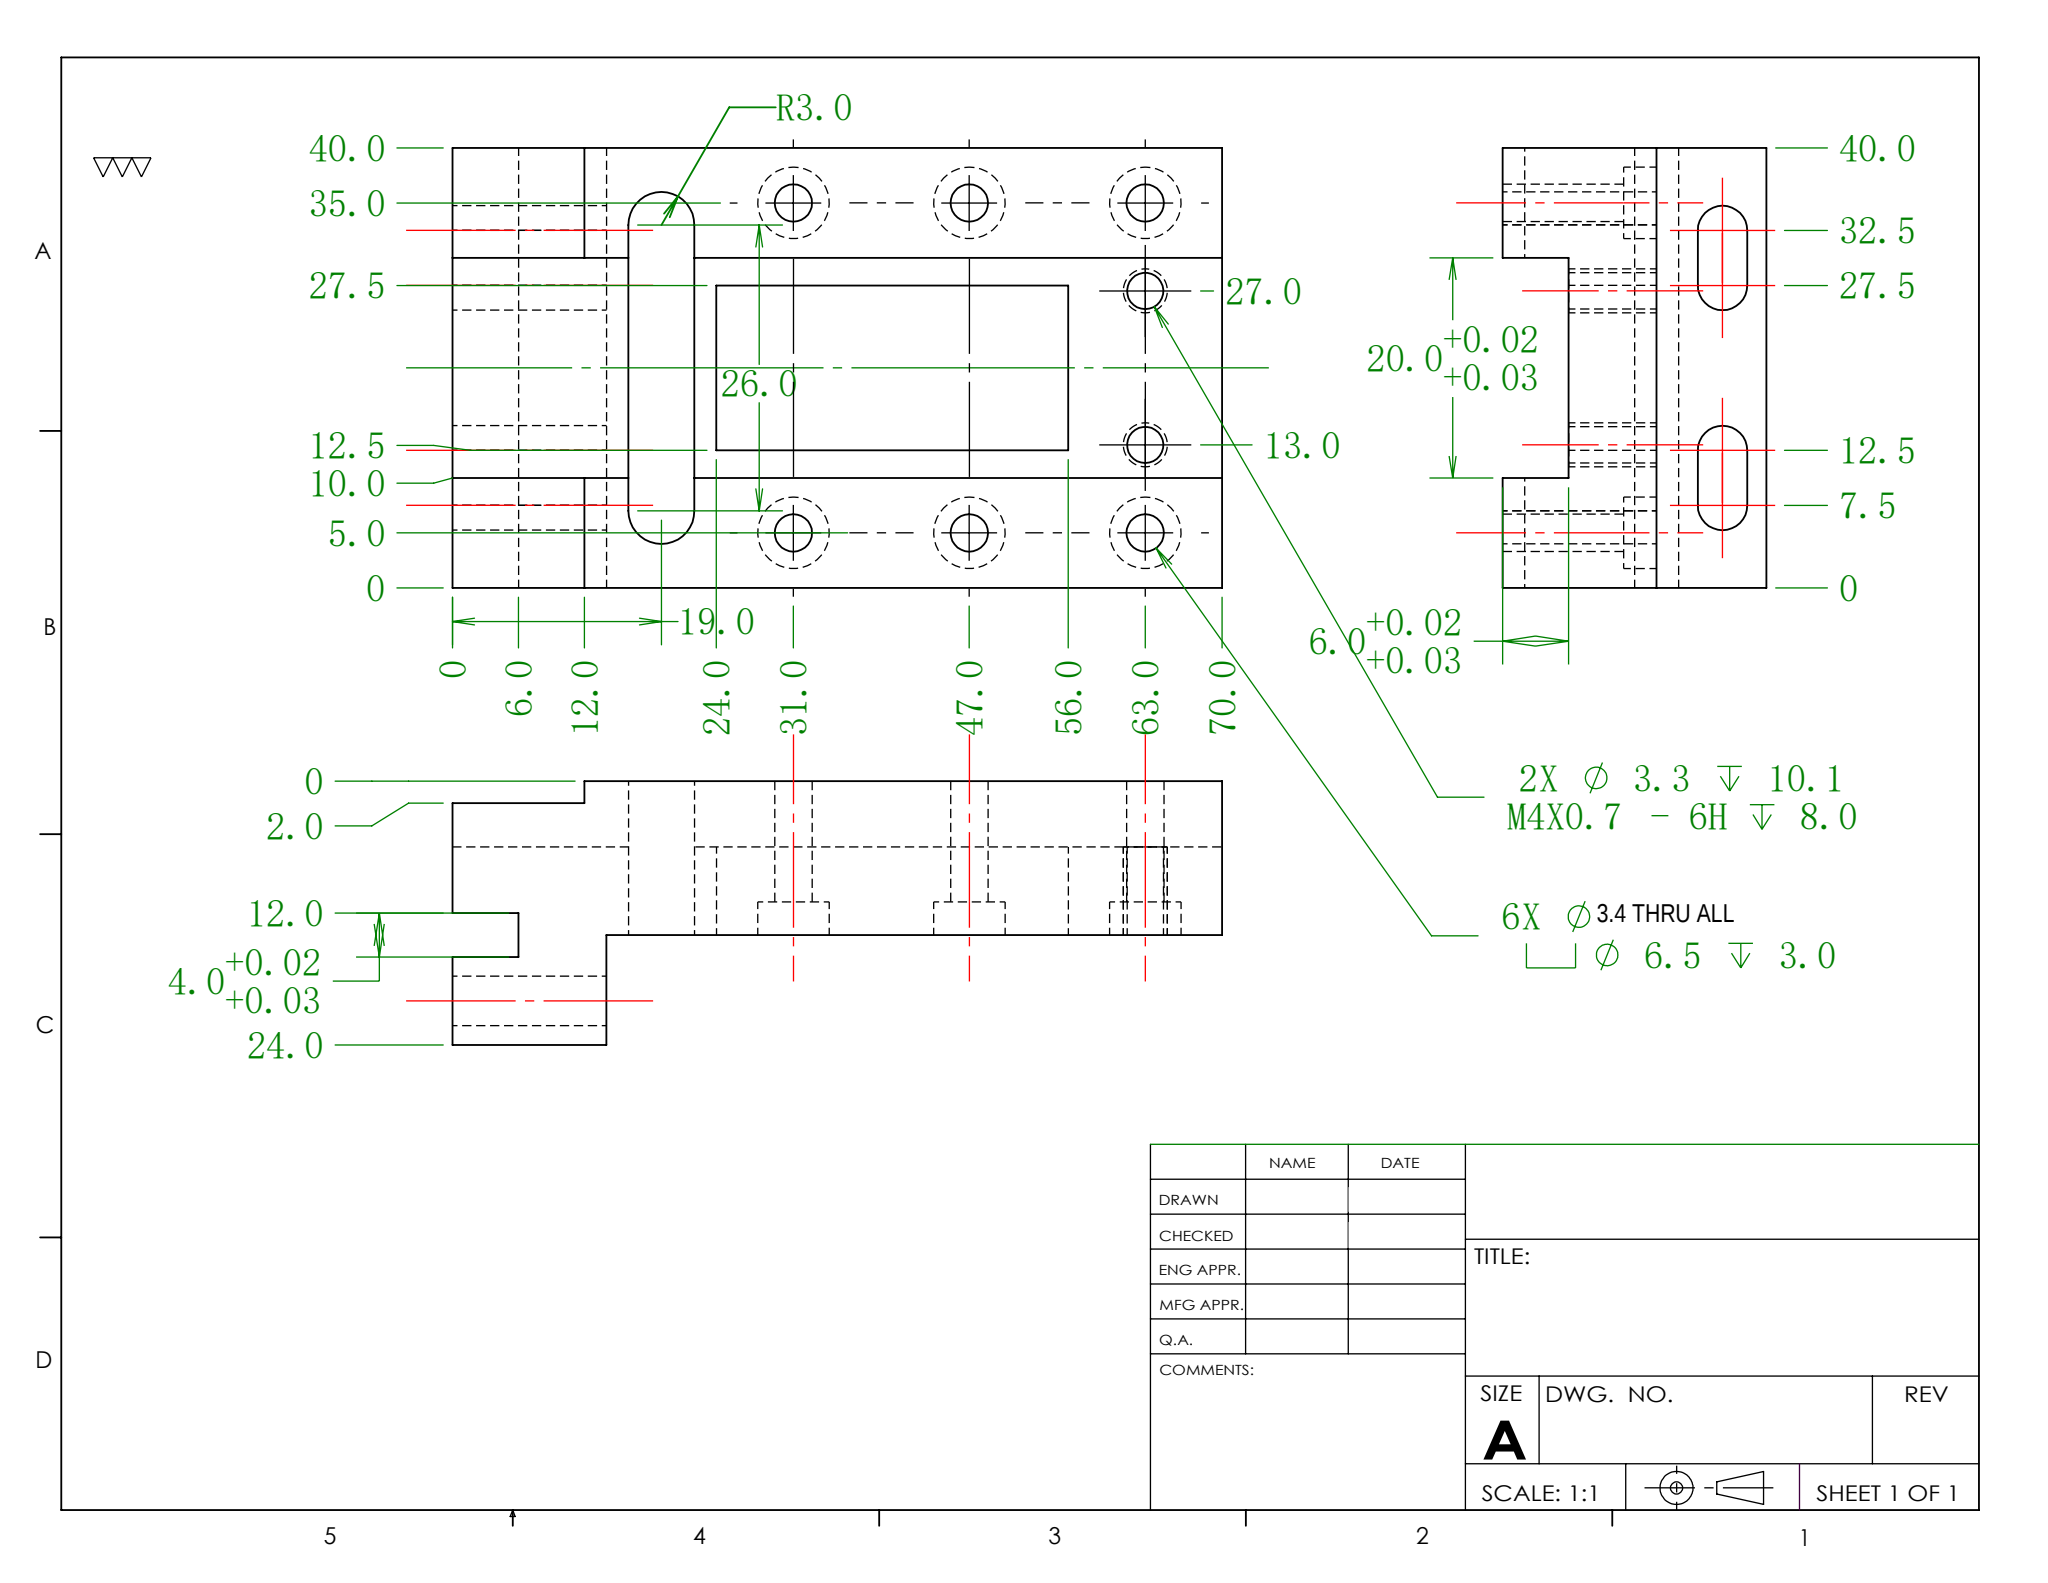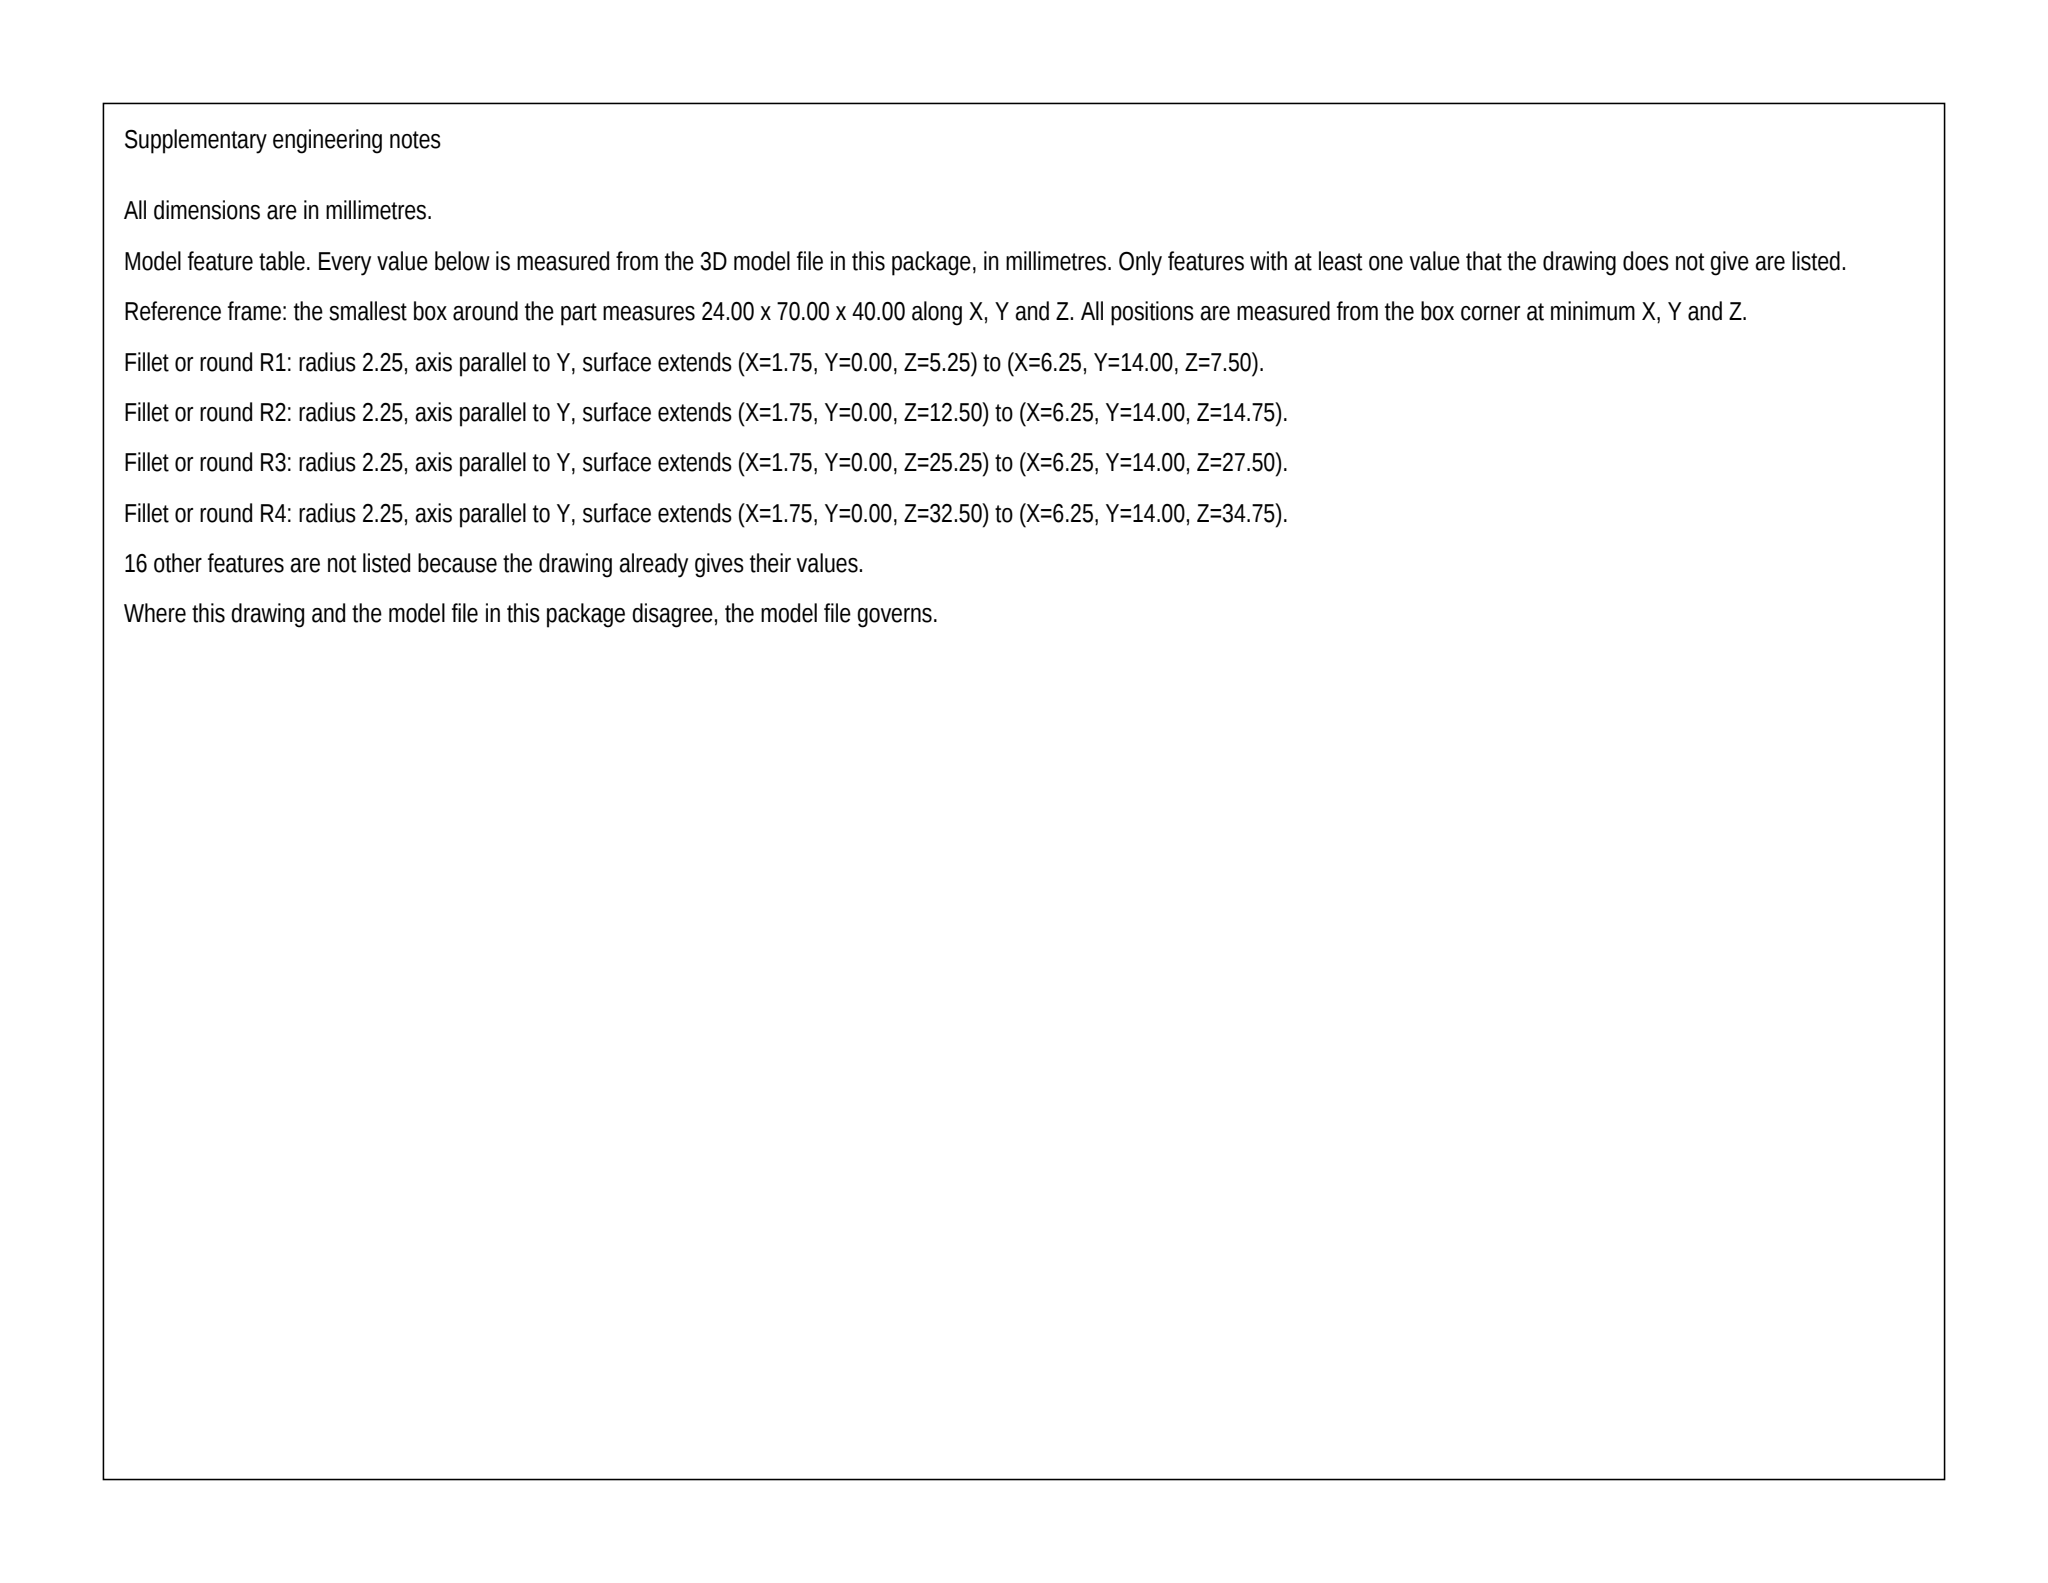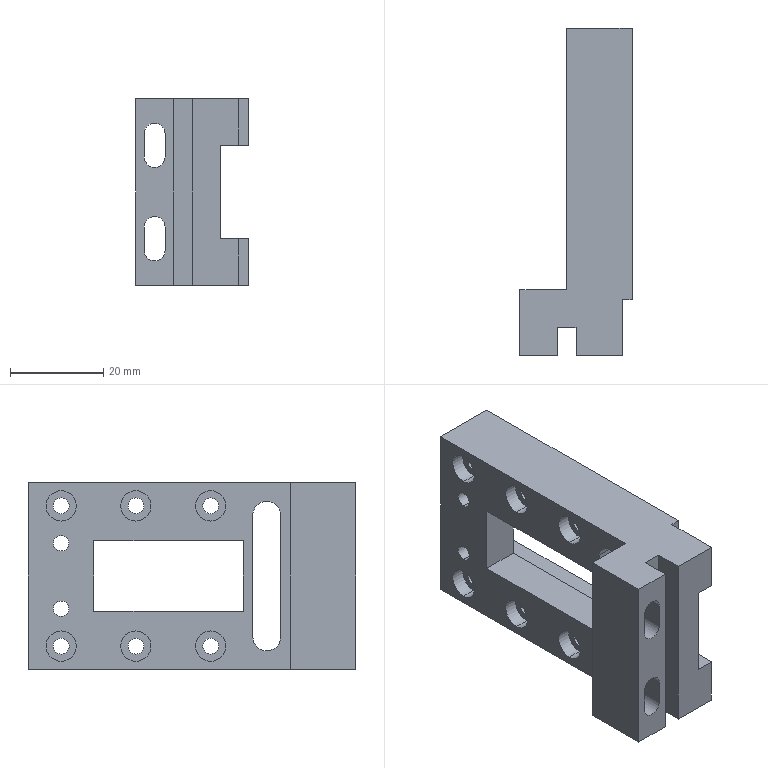Part | SolidWorks | mm | 1 solid | 76 faces | box 24 x 70 x 40 mm | volume 26851 mm3 | plane 39 | cylinder 37 | commonest cylinder face diameters 6.5 x12 3.4 x12 4.5 x6 3.3 x4 6 x3
build123d program:
from build123d import *

# Parameters (mm, degrees)
SKETCH1_W                                            = 40
SKETCH1_H                                            = 70
EXTRUDE1_DEPTH                                       = 12
SKETCH2_W                                            = 20
SKETCH2_H                                            = 80
EXTRUDE2_DEPTH                                       = 6
SKETCH3_W                                            = 40
SKETCH3_H                                            = 14
EXTRUDE3_DEPTH                                       = 12
SKETCH4_W                                            = 4
SKETCH4_H                                            = 6
EXTRUDE4_DEPTH                                       = 82.511
EXTRUDE5_DEPTH                                       = 70.857
SKETCH12_W                                           = 40
SKETCH12_H                                           = 56
EXTRUDE6_DEPTH                                       = 2
CYLINDRICAL_COUNTERSUNK_HOLE_FOR_M3_SOCK_D           = 3.4
CYLINDRICAL_COUNTERSUNK_HOLE_FOR_M3_SOCK_CBORE_D     = 6.5
CYLINDRICAL_COUNTERSUNK_HOLE_FOR_M3_SOCK_CBORE_DEPTH = 3
LPATTERN1_COUNT                                      = 2
LPATTERN1_PITCH                                      = 30
LPATTERN1_COUNT_DIR2                                 = 3
LPATTERN1_PITCH_DIR2                                 = 16
M4X0_7_TAPPED_HOLE1_D                                = 3.3
M4X0_7_TAPPED_HOLE1_DEPTH                            = 10.1
M4X0_7_TAPPED_HOLE1_TIP                              = 0.9914
SKETCH17_W                                           = 15
SKETCH17_H                                           = 28
EXTRUDE7_DEPTH                                       = 82.829
SKETCH18_W                                           = 8
SKETCH18_H                                           = 15
EXTRUDE8_DEPTH                                       = 4
SKETCH19_W                                           = 40
SKETCH19_H                                           = 12
EXTRUDE9_DEPTH                                       = 2
CUT_EXTRUDE1_DEPTH                                   = 82.829


with BuildPart() as part:
    # Sketch1 → Extrude1 (new body)
    with BuildSketch(Plane(origin=(0, 0, 0), x_dir=(0, 0, -1), z_dir=(1, 0, 0))):
        with Locations((20, 35)):
            Rectangle(SKETCH1_W, SKETCH1_H)
    extrude(amount=EXTRUDE1_DEPTH)

    # Sketch2 → Extrude2 (cut)
    with BuildSketch(Plane(origin=(12, 0, 0), x_dir=(0, 0, -1), z_dir=(1, 0, 0))):
        with Locations((20, 30)):
            Rectangle(SKETCH2_W, SKETCH2_H)
    extrude(amount=-EXTRUDE2_DEPTH, mode=Mode.SUBTRACT)

    # Sketch3 → Extrude3 (add)
    with BuildSketch(Plane.ZY):
        with Locations((-20, 7)):
            Rectangle(SKETCH3_W, SKETCH3_H)
    extrude(amount=EXTRUDE3_DEPTH)

    # Sketch4 → Extrude4 (cut, through all)
    with BuildSketch(Plane(origin=(0, 0, -40), x_dir=(-1, 0, 0), z_dir=(0, 0, -1))):
        with Locations((2, 3)):
            Rectangle(SKETCH4_W, SKETCH4_H)
    extrude(amount=-EXTRUDE4_DEPTH, mode=Mode.SUBTRACT)

    # Sketch5 → Extrude5 (cut, through all)
    with BuildSketch(Plane(origin=(0, 14, 0), x_dir=(1, 0, 0), z_dir=(0, 1, 0))):
        with BuildLine():
            Line((-5.75, 32.5), (-5.75, 27.5))
            ThreePointArc((-5.75, 27.5), (-8, 25.25), (-10.25, 27.5))
            Line((-10.25, 27.5), (-10.25, 32.5))
            ThreePointArc((-10.25, 32.5), (-8, 34.75), (-5.75, 32.5))
        make_face()
        with BuildLine():
            Line((-5.75, 12.5), (-5.75, 7.5))
            ThreePointArc((-5.75, 7.5), (-8, 5.25), (-10.25, 7.5))
            Line((-10.25, 7.5), (-10.25, 12.5))
            ThreePointArc((-10.25, 12.5), (-8, 14.75), (-5.75, 12.5))
        make_face()
    extrude(amount=-EXTRUDE5_DEPTH, mode=Mode.SUBTRACT)

    # Sketch12 → Extrude6 (add)
    with BuildSketch(Plane.ZY):
        with Locations((-20, 42)):
            Rectangle(SKETCH12_W, SKETCH12_H)
    extrude(amount=EXTRUDE6_DEPTH)

    # Cylindrical Countersunk Hole for M3 Sock (through all)
    with Locations(Plane.ZY.offset(2)):
        with Locations((-35, 63)):
            cylindrical_countersunk_hole_for_m3_sock = CounterBoreHole(CYLINDRICAL_COUNTERSUNK_HOLE_FOR_M3_SOCK_D / 2, CYLINDRICAL_COUNTERSUNK_HOLE_FOR_M3_SOCK_CBORE_D / 2, CYLINDRICAL_COUNTERSUNK_HOLE_FOR_M3_SOCK_CBORE_DEPTH)

    # LPattern1: Cylindrical Countersunk Hole for M3 Sock 2 × 3
    with Locations(*[(0, -j * LPATTERN1_PITCH_DIR2, i * LPATTERN1_PITCH) for i in range(LPATTERN1_COUNT) for j in range(LPATTERN1_COUNT_DIR2) if (i, j) != (0, 0)]):
        add(cylindrical_countersunk_hole_for_m3_sock, mode=Mode.SUBTRACT)

    # M4x0.7 Tapped Hole1
    with Locations(Plane.ZY.offset(2)):
        with Locations((-27, 63), (-13, 63)):
            Hole(M4X0_7_TAPPED_HOLE1_D / 2, depth=M4X0_7_TAPPED_HOLE1_DEPTH)
            with Locations((0, 0, -(M4X0_7_TAPPED_HOLE1_DEPTH + M4X0_7_TAPPED_HOLE1_TIP / 2))):  # 118° drill point
                Cone(0, M4X0_7_TAPPED_HOLE1_D / 2, M4X0_7_TAPPED_HOLE1_TIP, mode=Mode.SUBTRACT)

    # Sketch17 → Extrude7 (cut, through all)
    with BuildSketch(Plane.ZY.offset(2)):
        with Locations((-20, 42)):
            Rectangle(SKETCH17_W, SKETCH17_H)
    extrude(amount=-EXTRUDE7_DEPTH, mode=Mode.SUBTRACT)

    # Sketch18 → Extrude8 (cut)
    with BuildSketch(Plane(origin=(0, 28, 0), x_dir=(1, 0, 0), z_dir=(0, 1, 0))):
        with Locations((2, 20)):
            Rectangle(SKETCH18_W, SKETCH18_H)
    extrude(amount=-EXTRUDE8_DEPTH, mode=Mode.SUBTRACT)

    # Sketch19 → Extrude9 (cut)
    with BuildSketch(Plane(origin=(12, 0, 0), x_dir=(0, 0, -1), z_dir=(1, 0, 0))):
        with Locations((20, 6)):
            Rectangle(SKETCH19_W, SKETCH19_H)
    extrude(amount=-EXTRUDE9_DEPTH, mode=Mode.SUBTRACT)

    # Sketch20 → Cut-Extrude1 (cut, through all)
    with BuildSketch(Plane.ZY.offset(2)):
        with BuildLine():
            Line((-33, 22), (-7, 22))
            ThreePointArc((-7, 22), (-4, 19), (-7, 16))
            Line((-7, 16), (-33, 16))
            ThreePointArc((-33, 16), (-36, 19), (-33, 22))
        make_face()
    extrude(amount=-CUT_EXTRUDE1_DEPTH, mode=Mode.SUBTRACT)


solid = part.part